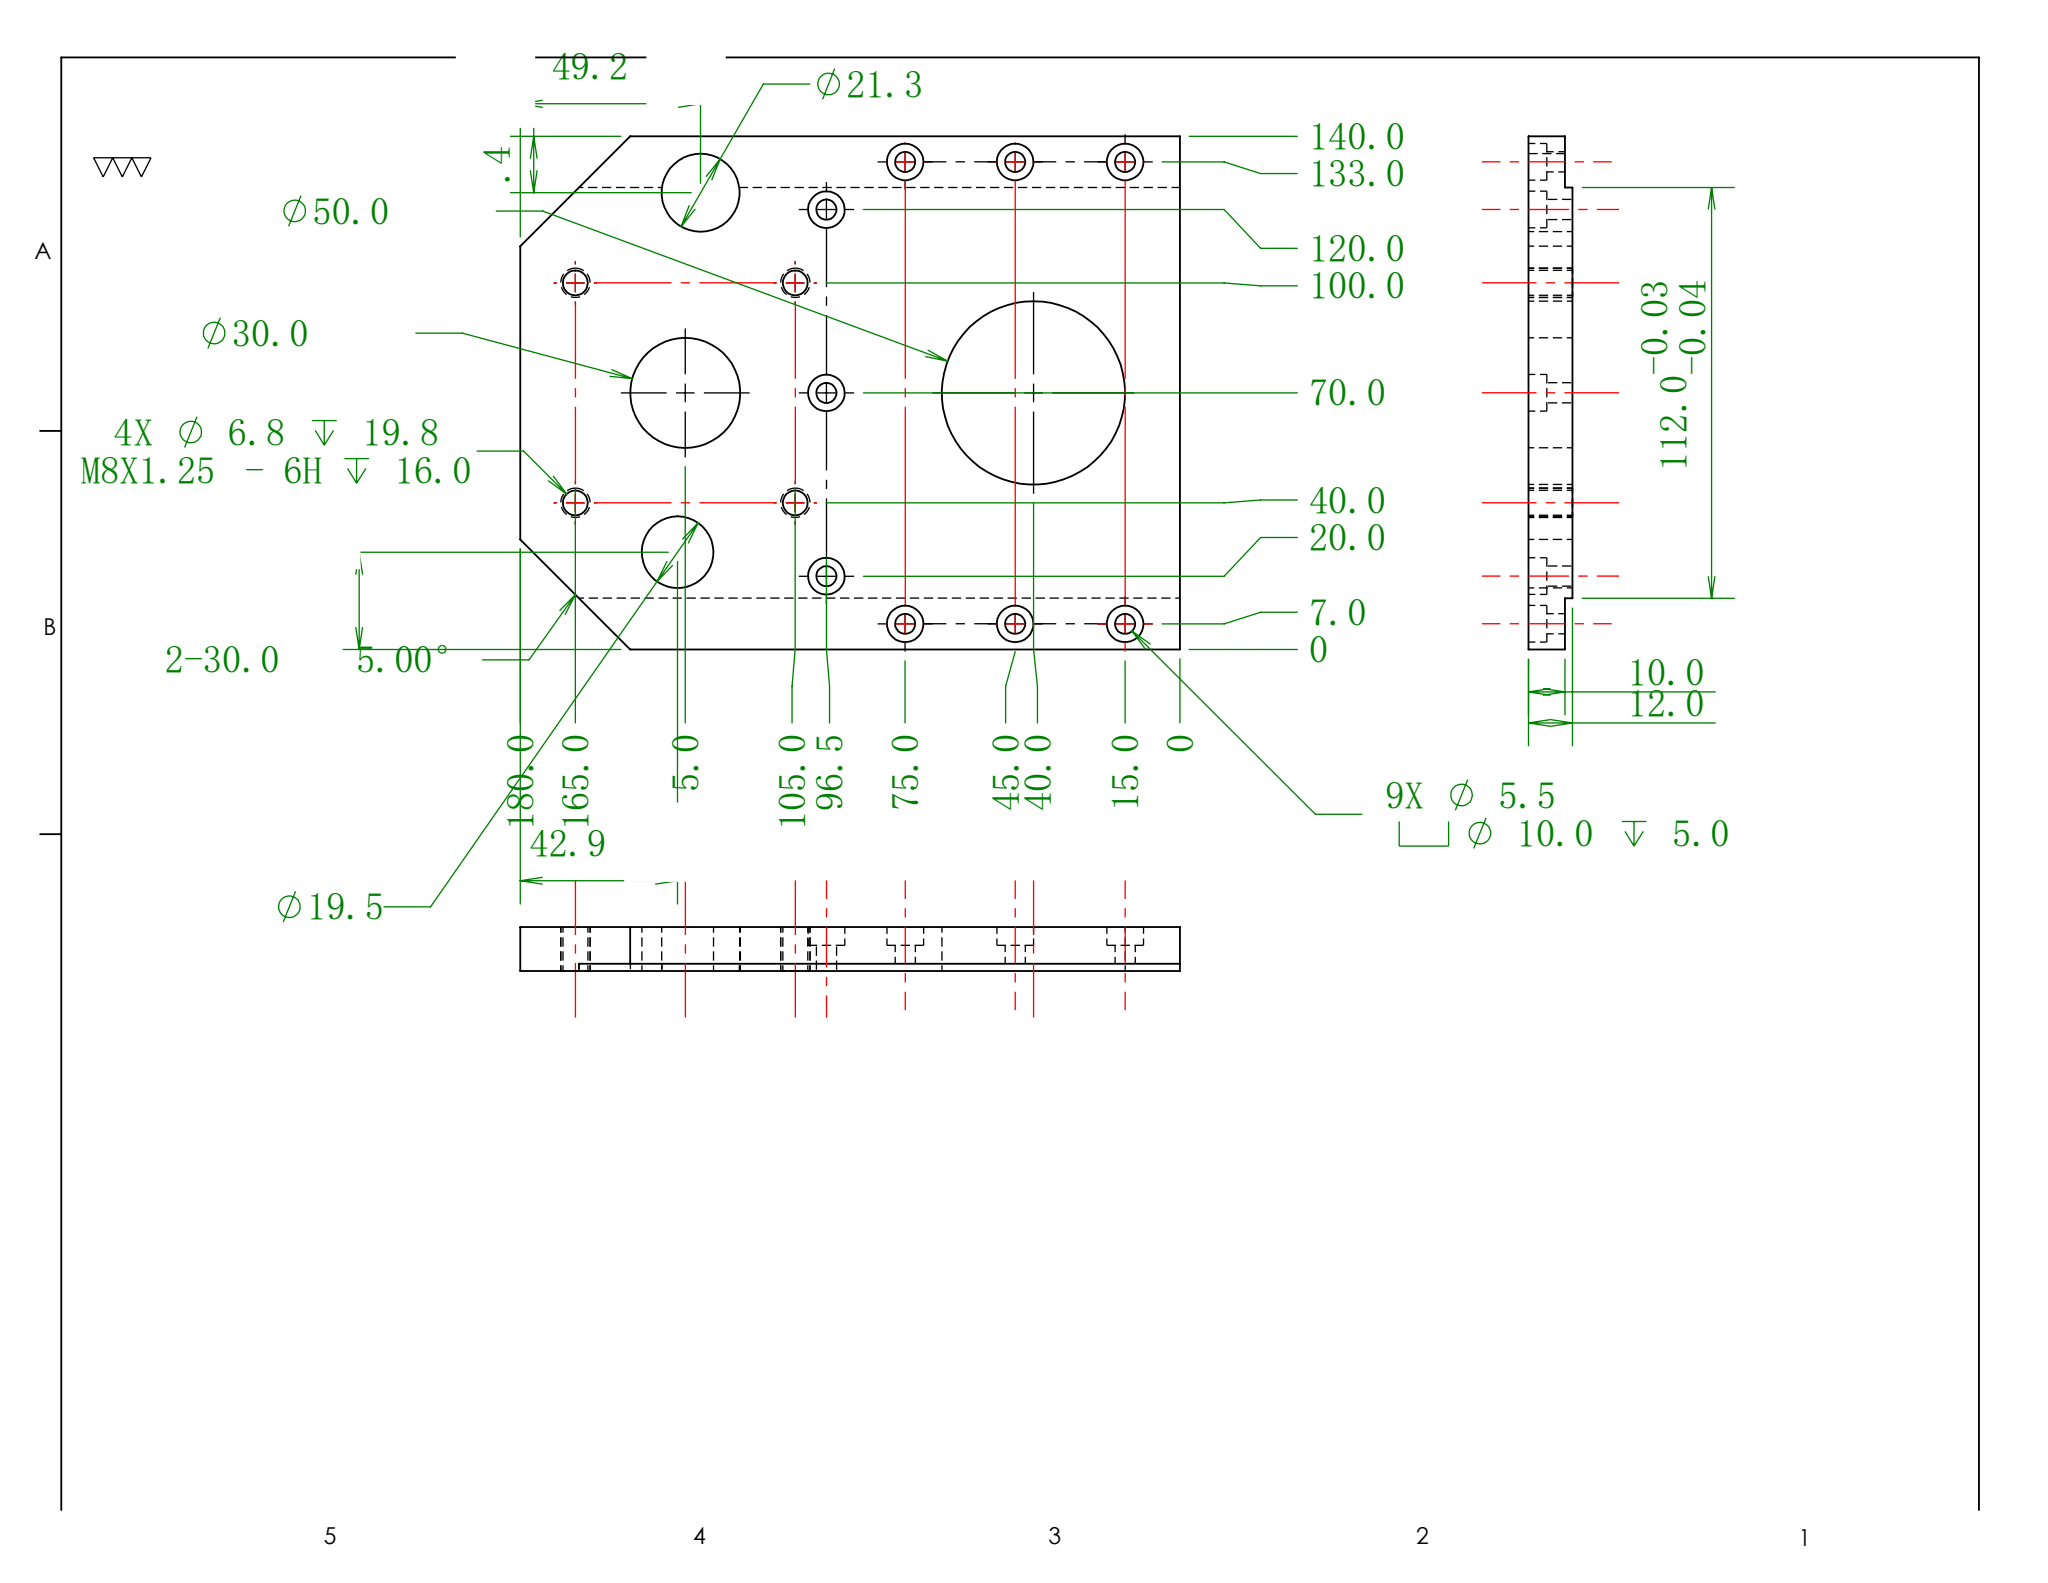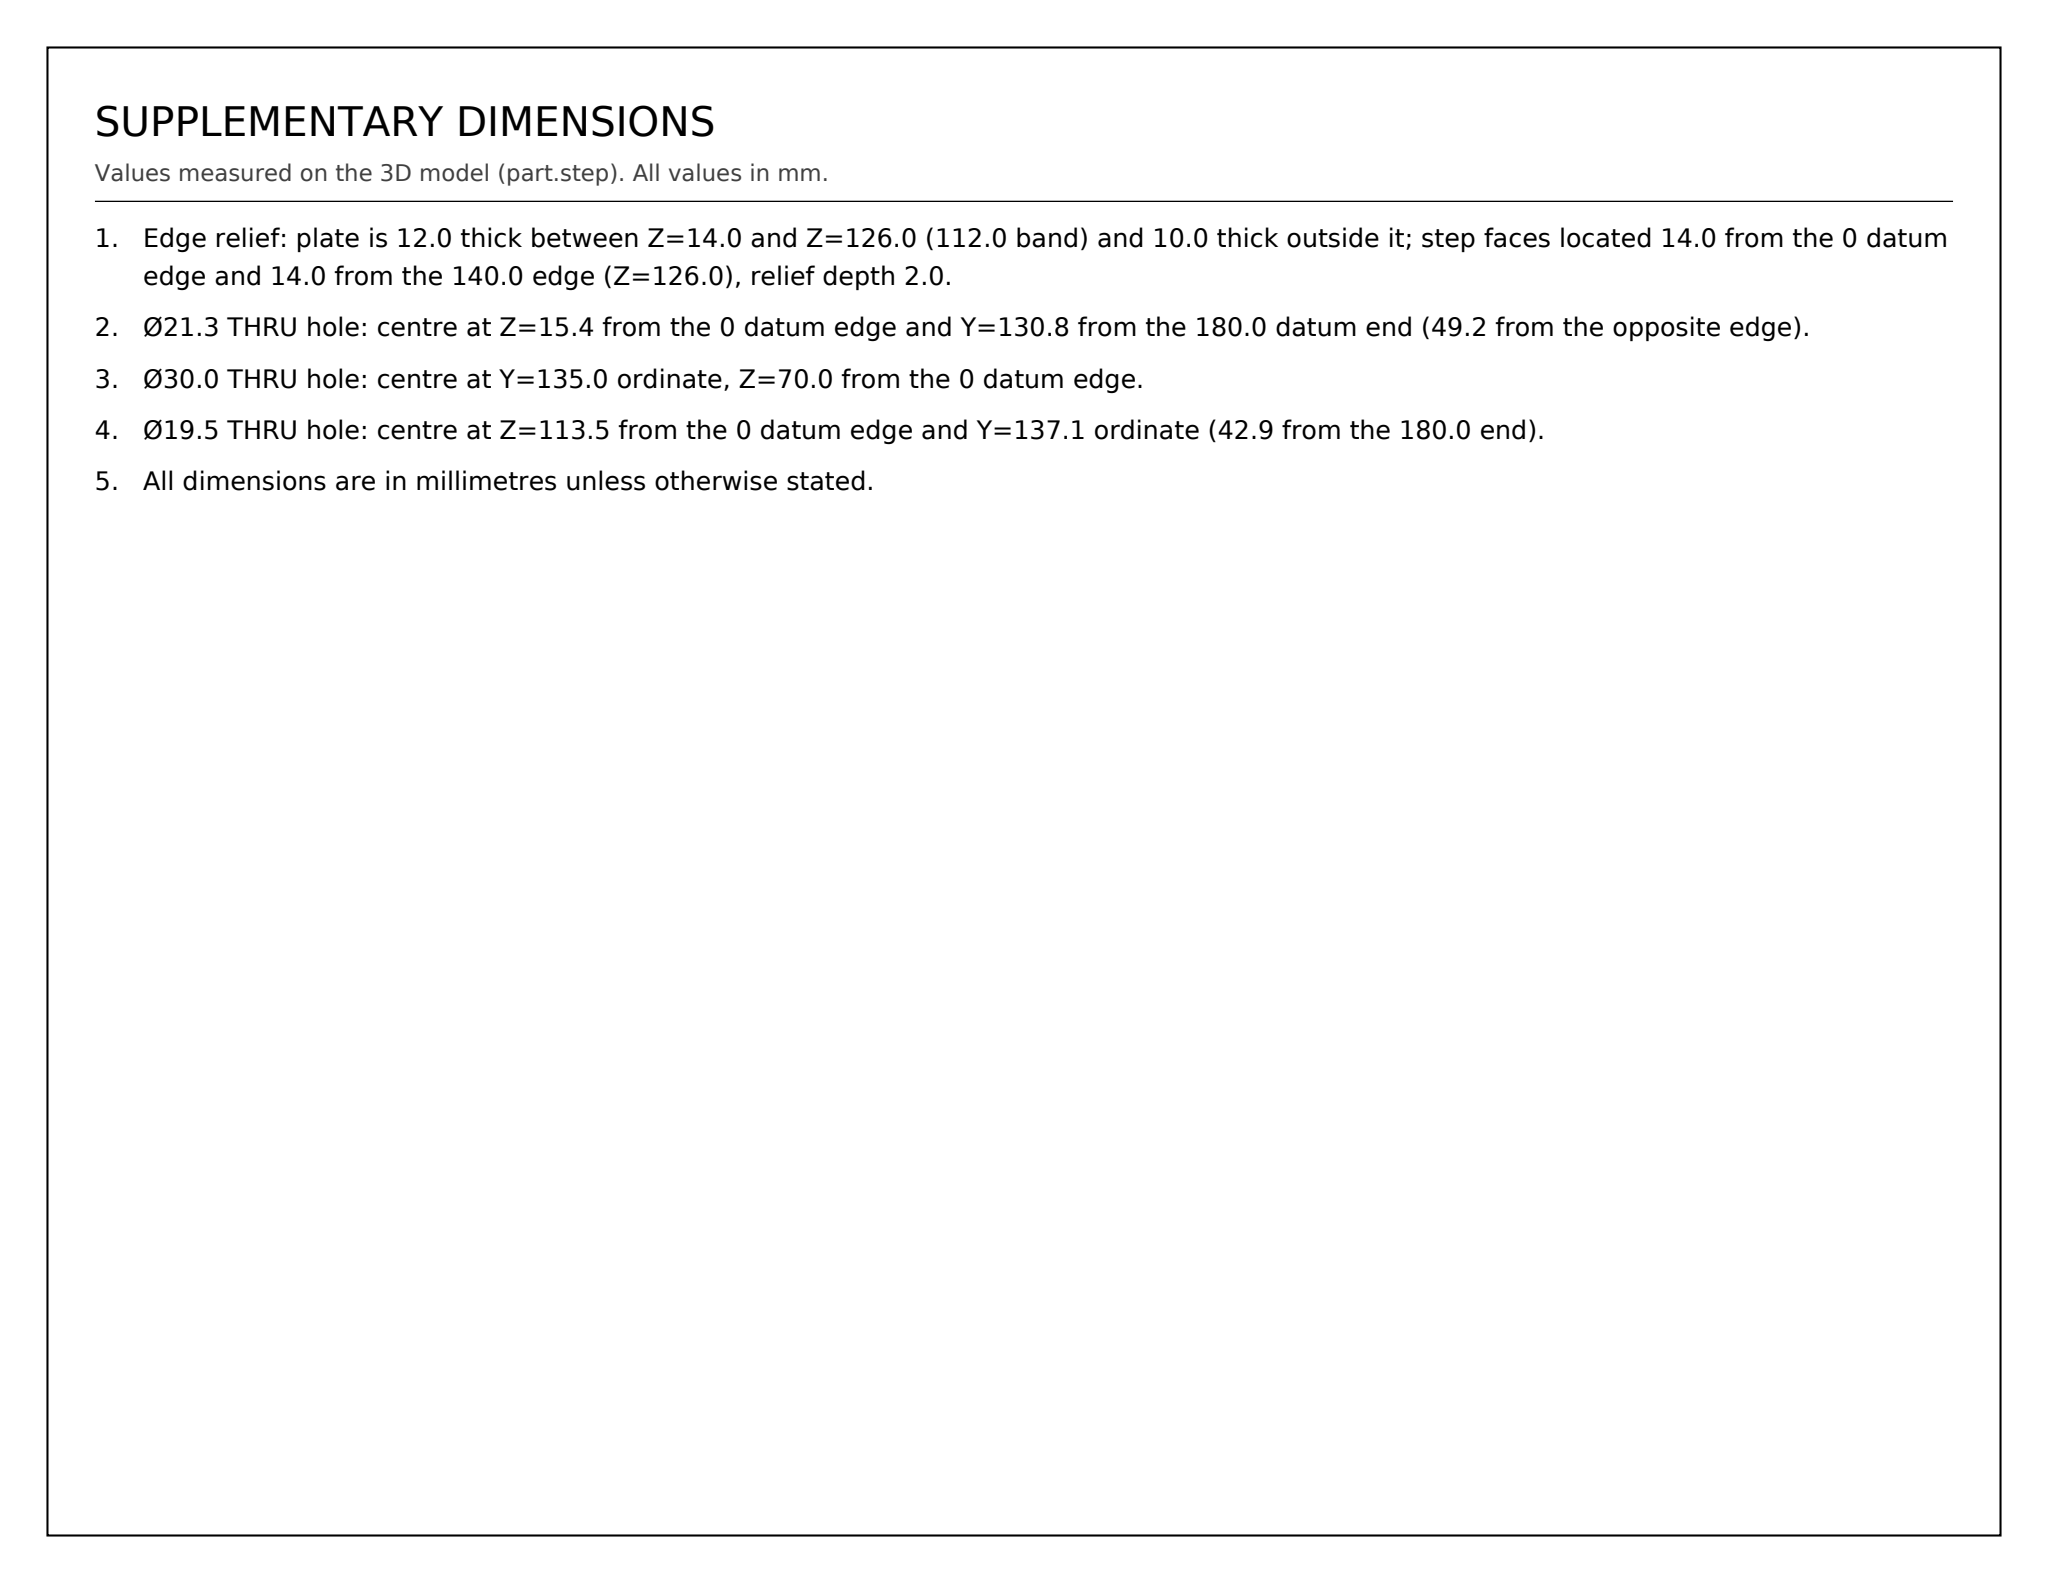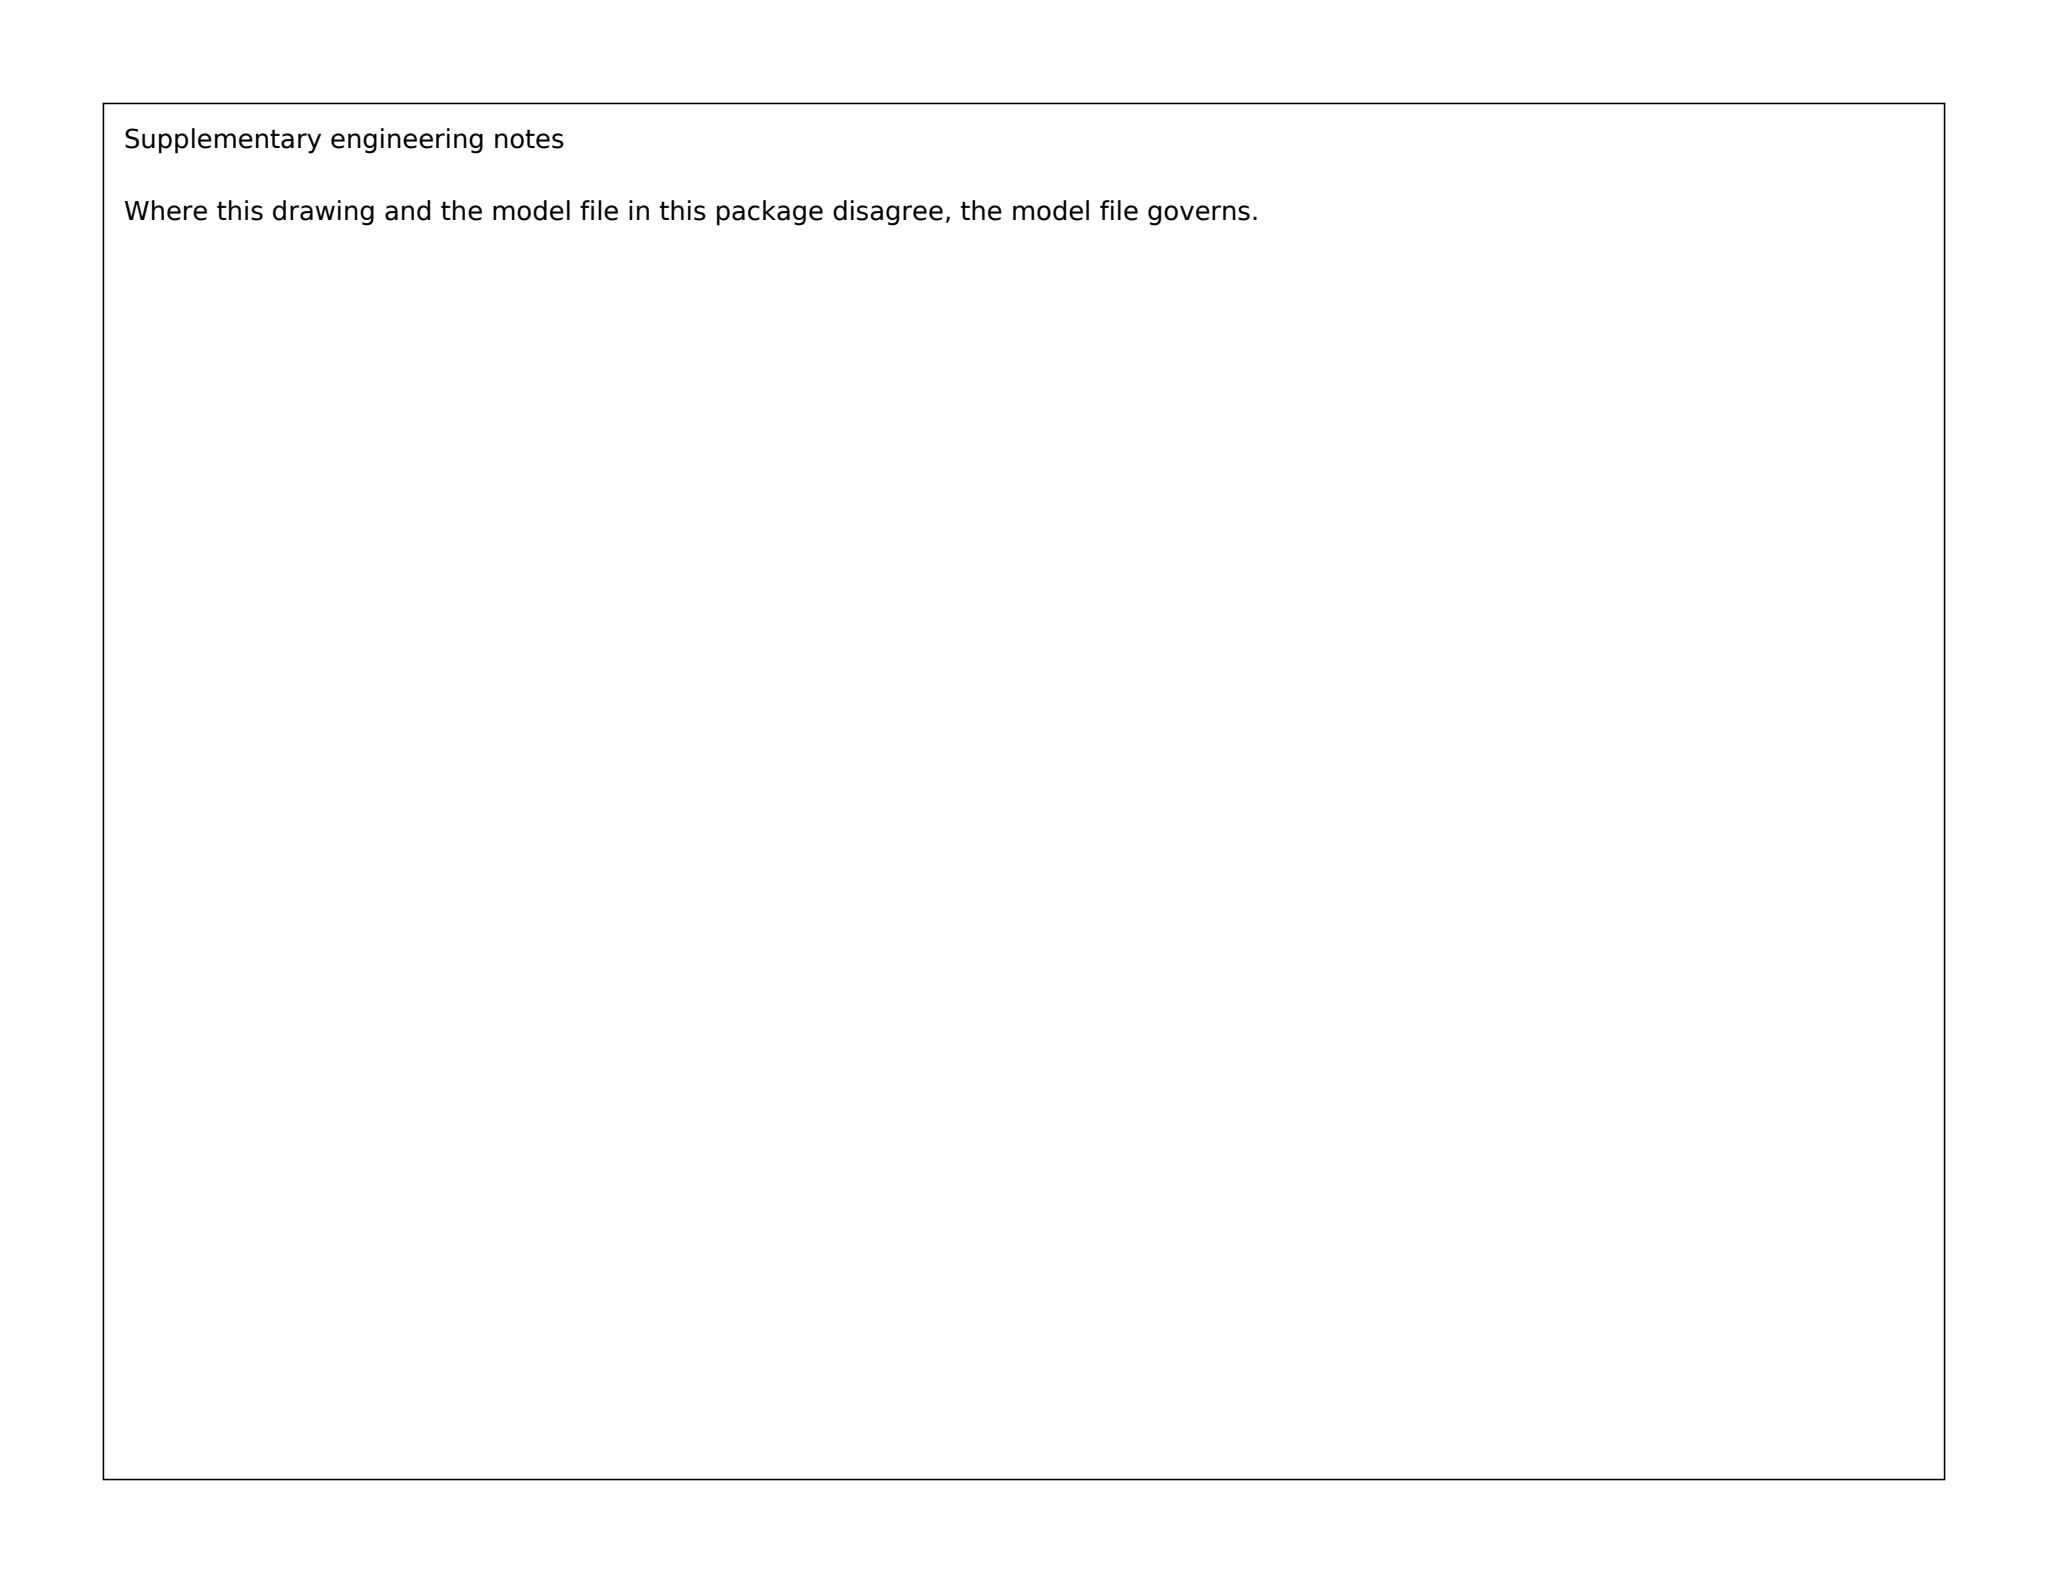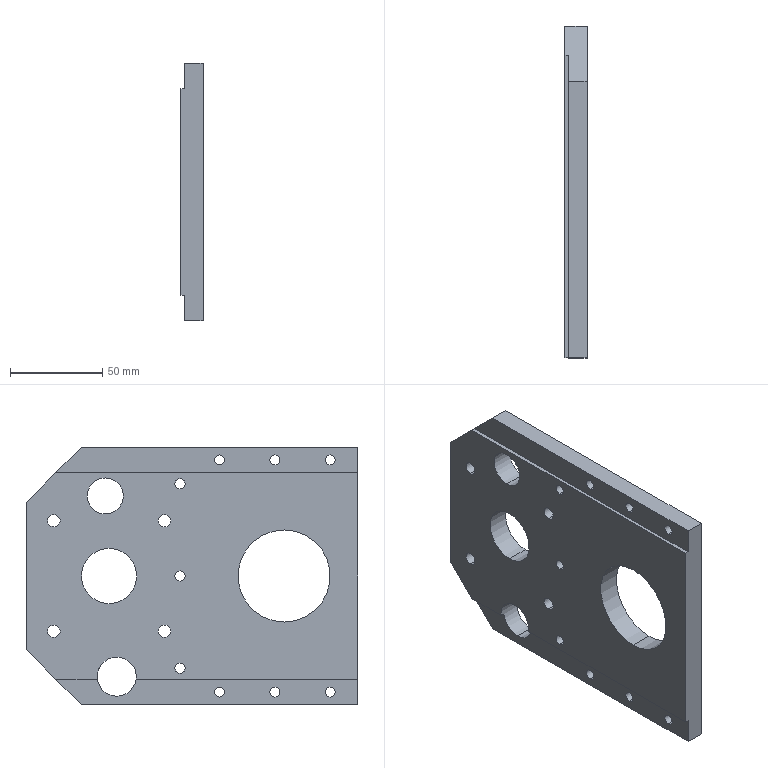Part | SolidWorks | mm | 1 solid | 74 faces | box 12 x 180 x 140 mm | volume 236708 mm3 | cylinder 52 | plane 22 | commonest cylinder face diameters 5.5 x18 10 x18 6.8 x8 19.538 x2 21.273 x2 50 x2 30 x2
Drawing notes:
Edge relief: plate is 12.0 thick between Z=14.0 and Z=126.0 (112.0 band) and 10.0 thick outside it; step faces located 14.0 from the 0 datum edge and 14.0 from the 140.0 edge (Z=126.0), relief depth 2.0. | from the solid: axis_planes z=14.0 and z=126.0 with x-planes at 2.0 and 12.0 (bbox_xyz x=12.0)
Ø21.3 THRU hole: centre at Z=15.4 from the 0 datum edge and Y=130.8 from the 180.0 datum end (49.2 from the opposite edge). | from the solid: cylinders [21.273, axis x, pos [null,130.83,15.39], length 12.0]
Ø30.0 THRU hole: centre at Y=135.0 ordinate, Z=70.0 from the 0 datum edge. | from the solid: cylinders [30.0, axis x, pos [null,135.0,70.0], length 12.0]
Ø19.5 THRU hole: centre at Z=113.5 from the 0 datum edge and Y=137.1 ordinate (42.9 from the 180.0 end). | from the solid: cylinders [19.538, axis x, pos [null,137.09,113.45], length 12.0]
All dimensions are in millimetres unless otherwise stated. | from the solid: STEP model units mm, bbox_xyz 12.0 x 180.0 x 140.0
build123d program:
from build123d import *

# Parameters (mm, degrees)
SKETCH1_W                                       = 140
SKETCH1_H                                       = 180
EXTRUDE1_DEPTH                                  = 12
SKETCH2_R                                       = 15
EXTRUDE2_DEPTH                                  = 229.351
CHAMFER1_SIZE                                   = 30
SKETCH3_R                                       = 25
EXTRUDE3_DEPTH                                  = 229.351
SKETCH4_W                                       = 14
SKETCH4_H                                       = 180
CUT_EXTRUDE1_DEPTH                              = 2
M5_HEX_SOCKET_HEAD_CAP_SCREW_CBORE1_D           = 5.5
M5_HEX_SOCKET_HEAD_CAP_SCREW_CBORE1_CBORE_D     = 10
M5_HEX_SOCKET_HEAD_CAP_SCREW_CBORE1_CBORE_DEPTH = 5
LPATTERN1_COUNT                                 = 3
LPATTERN1_PITCH                                 = 30
M5_HEX_SOCKET_HEAD_CAP_SCREW_CBORE2_D           = 5.5
M5_HEX_SOCKET_HEAD_CAP_SCREW_CBORE2_CBORE_D     = 10
M5_HEX_SOCKET_HEAD_CAP_SCREW_CBORE2_CBORE_DEPTH = 5
LPATTERN2_COUNT                                 = 3
LPATTERN2_PITCH                                 = 50
M8X1_25_TAPPED_HOLE1_D                          = 6.8
M8X1_25_TAPPED_HOLE1_DEPTH                      = 19.75
M8X1_25_TAPPED_HOLE1_TIP                        = 2.043
SKETCH11_R                                      = 9.769
SKETCH11_R_2                                    = 10.636
CUT_EXTRUDE2_DEPTH                              = 68


with BuildPart() as part:
    # Sketch1 → Extrude1 (new body)
    with BuildSketch(Plane(origin=(0, 0, 0), x_dir=(0, 0, -1), z_dir=(1, 0, 0))):
        with Locations((70, 90)):
            Rectangle(SKETCH1_W, SKETCH1_H)
    extrude(amount=EXTRUDE1_DEPTH)

    # Sketch2 → Extrude2 (cut, through all)
    with BuildSketch(Plane(origin=(12, 0, 0), x_dir=(0, 0, -1), z_dir=(1, 0, 0))):
        with Locations((70, 135)):
            Circle(SKETCH2_R)
    extrude(amount=-EXTRUDE2_DEPTH, mode=Mode.SUBTRACT)

    # Chamfer1
    chamfer1_edges = [part.edges().sort_by_distance(p)[0] for p in [
        (6, 180, 0),
        (6, 180, -140),
    ]]
    chamfer(chamfer1_edges, length=CHAMFER1_SIZE)

    # Sketch3 → Extrude3 (cut, through all)
    with BuildSketch(Plane(origin=(12, 0, 0), x_dir=(0, 0, -1), z_dir=(1, 0, 0))):
        with Locations((70, 40)):
            Circle(SKETCH3_R)
    extrude(amount=-EXTRUDE3_DEPTH, mode=Mode.SUBTRACT)

    # Sketch4 → Cut-Extrude1 (cut)
    with BuildSketch(Plane.ZY):
        with Locations((-133, 90)):
            Rectangle(SKETCH4_W, SKETCH4_H)
        with Locations((-7, 90)):
            Rectangle(SKETCH4_W, SKETCH4_H)
    extrude(amount=-CUT_EXTRUDE1_DEPTH, mode=Mode.SUBTRACT)

    # M5 Hex Socket Head Cap Screw CBORE1 (through all)
    with Locations(Plane(origin=(12, 0, 0), x_dir=(0, 0, -1), z_dir=(1, 0, 0))):
        with Locations((7, 15), (133, 15)):
            m5_hex_socket_head_cap_screw_cbore1 = CounterBoreHole(M5_HEX_SOCKET_HEAD_CAP_SCREW_CBORE1_D / 2, M5_HEX_SOCKET_HEAD_CAP_SCREW_CBORE1_CBORE_D / 2, M5_HEX_SOCKET_HEAD_CAP_SCREW_CBORE1_CBORE_DEPTH)

    # LPattern1: M5 Hex Socket Head Cap Screw CBORE1 ×3
    with Locations(*[(0, i * LPATTERN1_PITCH, 0) for i in range(1, LPATTERN1_COUNT)]):
        add(m5_hex_socket_head_cap_screw_cbore1, mode=Mode.SUBTRACT)

    # M5 Hex Socket Head Cap Screw CBORE2 (through all)
    with Locations(Plane(origin=(12, 0, 0), x_dir=(0, 0, -1), z_dir=(1, 0, 0))):
        with Locations((20, 96.5)):
            m5_hex_socket_head_cap_screw_cbore2 = CounterBoreHole(M5_HEX_SOCKET_HEAD_CAP_SCREW_CBORE2_D / 2, M5_HEX_SOCKET_HEAD_CAP_SCREW_CBORE2_CBORE_D / 2, M5_HEX_SOCKET_HEAD_CAP_SCREW_CBORE2_CBORE_DEPTH)

    # LPattern2: M5 Hex Socket Head Cap Screw CBORE2 ×3
    with Locations(*[(0, 0, -i * LPATTERN2_PITCH) for i in range(1, LPATTERN2_COUNT)]):
        add(m5_hex_socket_head_cap_screw_cbore2, mode=Mode.SUBTRACT)

    # M8x1.25 Tapped Hole1
    with Locations(Plane(origin=(12, 0, 0), x_dir=(0, 0, -1), z_dir=(1, 0, 0))):
        with Locations((40, 165), (100, 165), (100, 105), (40, 105)):
            Hole(M8X1_25_TAPPED_HOLE1_D / 2, depth=M8X1_25_TAPPED_HOLE1_DEPTH)
            with Locations((0, 0, -(M8X1_25_TAPPED_HOLE1_DEPTH + M8X1_25_TAPPED_HOLE1_TIP / 2))):  # 118° drill point
                Cone(0, M8X1_25_TAPPED_HOLE1_D / 2, M8X1_25_TAPPED_HOLE1_TIP, mode=Mode.SUBTRACT)

    # Sketch11 → Cut-Extrude2 (cut)
    with BuildSketch(Plane(origin=(12, 0, 0), x_dir=(0, 0, -1), z_dir=(1, 0, 0))):
        with Locations((26.547, 137.094)):
            Circle(SKETCH11_R)
        with Locations((124.606, 130.827)):
            Circle(SKETCH11_R_2)
    extrude(amount=-CUT_EXTRUDE2_DEPTH, mode=Mode.SUBTRACT)


solid = part.part